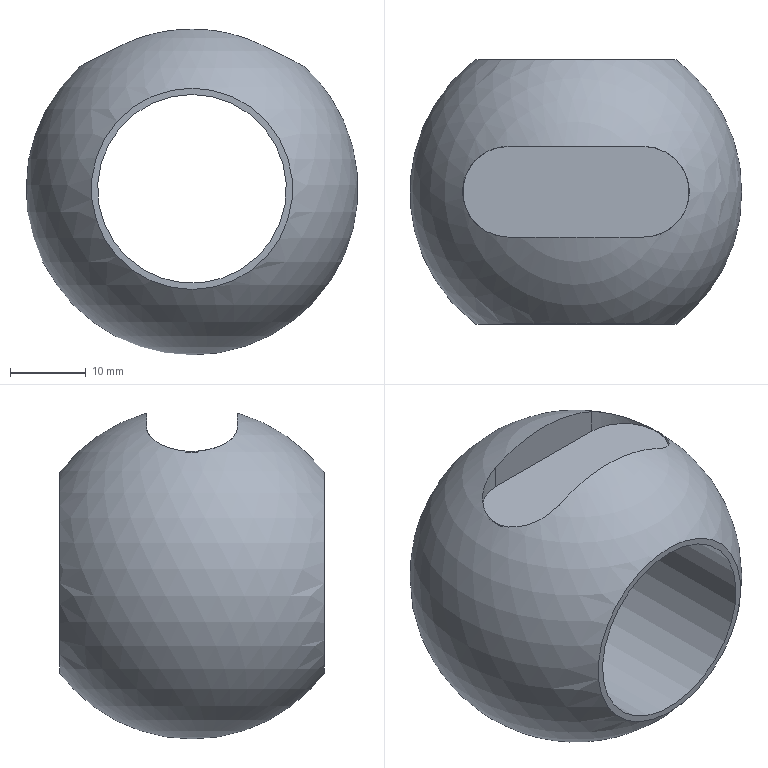Component | NX | VALVECORE | 1 solid | 9 faces | box 44 x 35 x 43.17 mm | volume 23444 mm3 | plane 5 | cylinder 3 | sphere 1 | commonest cylinder face diameters 12 x2 25 x1
STEP:
#1=CARTESIAN_POINT('',(0.,0.,0.));
#2=DIRECTION('',(0.,0.,1.));
#3=DIRECTION('',(1.,0.,0.));
#4=AXIS2_PLACEMENT_3D('',#1,#2,#3);
#5=CARTESIAN_POINT('',(186.165,20.5,51.157));
#6=VERTEX_POINT('',#5);
#7=CARTESIAN_POINT('',(168.165,20.5,51.157));
#8=VERTEX_POINT('',#7);
#9=CARTESIAN_POINT('',(177.165,20.5,32.));
#10=DIRECTION('',(0.,-1.,0.));
#11=DIRECTION('',(0.,0.,1.));
#12=AXIS2_PLACEMENT_3D('',#9,#10,#11);
#13=CIRCLE('',#12,21.166);
#14=CARTESIAN_POINT('',(177.165,26.5,32.));
#15=DIRECTION('',(0.,0.,1.));
#16=DIRECTION('',(1.,0.,0.));
#17=AXIS2_PLACEMENT_3D('',#14,#15,#16);
#18=SPHERICAL_SURFACE('',#17,22.);
#19=CARTESIAN_POINT('',(5.695,1.057));
#20=CARTESIAN_POINT('',(5.682,1.068));
#21=CARTESIAN_POINT('',(5.654,1.09));
#22=CARTESIAN_POINT('',(5.606,1.121));
#23=CARTESIAN_POINT('',(5.55,1.152));
#24=CARTESIAN_POINT('',(5.486,1.181));
#25=CARTESIAN_POINT('',(5.411,1.208));
#26=CARTESIAN_POINT('',(5.325,1.232));
#27=CARTESIAN_POINT('',(5.226,1.253));
#28=CARTESIAN_POINT('',(5.113,1.271));
#29=CARTESIAN_POINT('',(4.988,1.284));
#30=CARTESIAN_POINT('',(4.853,1.293));
#31=CARTESIAN_POINT('',(4.712,1.296));
#32=CARTESIAN_POINT('',(4.572,1.293));
#33=CARTESIAN_POINT('',(4.436,1.284));
#34=CARTESIAN_POINT('',(4.311,1.271));
#35=CARTESIAN_POINT('',(4.199,1.253));
#36=CARTESIAN_POINT('',(4.1,1.232));
#37=CARTESIAN_POINT('',(4.014,1.208));
#38=CARTESIAN_POINT('',(3.939,1.181));
#39=CARTESIAN_POINT('',(3.874,1.152));
#40=CARTESIAN_POINT('',(3.819,1.121));
#41=CARTESIAN_POINT('',(3.771,1.09));
#42=CARTESIAN_POINT('',(3.743,1.068));
#43=CARTESIAN_POINT('',(3.73,1.057));
#44=B_SPLINE_CURVE_WITH_KNOTS('',3,(#19,#20,#21,#22,#23,#24,#25,#26,#27,#28,#29,#30,#31,#32,#33,#34,#35,#36,#37,#38,#39,#40,#41,#42,#43),.UNSPECIFIED.,.F.,.F.,(4,1,1,1,1,1,1,1,1,1,1,1,1,1,1,1,1,1,1,1,1,1,4),(5.844,5.884,5.924,5.964,6.004,6.044,6.084,6.123,6.163,6.203,6.243,6.283,6.323,6.363,6.403,6.443,6.483,6.523,6.563,6.603,6.643,6.682,6.722),.QUASI_UNIFORM_KNOTS.);
#45=(GEOMETRIC_REPRESENTATION_CONTEXT(2)PARAMETRIC_REPRESENTATION_CONTEXT()REPRESENTATION_CONTEXT('',''));
#46=DEFINITIONAL_REPRESENTATION('',(#44),#45);
#47=PCURVE('',#18,#46);
#48=CARTESIAN_POINT('',(168.165,20.5,82.));
#49=DIRECTION('',(0.,1.,0.));
#50=DIRECTION('',(0.,0.,1.));
#51=AXIS2_PLACEMENT_3D('',#48,#49,#50);
#52=PLANE('',#51);
#53=CARTESIAN_POINT('',(-28.834,9.));
#54=CARTESIAN_POINT('',(-28.834,-27.661));
#55=CARTESIAN_POINT('',(-60.583,-9.33));
#56=CARTESIAN_POINT('',(-92.332,9.));
#57=CARTESIAN_POINT('',(-60.583,27.33));
#58=CARTESIAN_POINT('',(-28.834,45.661));
#59=CARTESIAN_POINT('',(-28.834,9.));
#60=(BOUNDED_CURVE()B_SPLINE_CURVE(2,(#53,#54,#55,#56,#57,#58,#59),.UNSPECIFIED.,.T.,.F.)B_SPLINE_CURVE_WITH_KNOTS((1,2,2,2,2,1),(-2.094,0.,2.094,4.189,6.283,8.378),.UNSPECIFIED.)CURVE()GEOMETRIC_REPRESENTATION_ITEM()RATIONAL_B_SPLINE_CURVE((1.,0.5,1.,0.5,1.,0.5,1.))REPRESENTATION_ITEM(''));
#61=(GEOMETRIC_REPRESENTATION_CONTEXT(2)PARAMETRIC_REPRESENTATION_CONTEXT()REPRESENTATION_CONTEXT('',''));
#62=DEFINITIONAL_REPRESENTATION('',(#60),#61);
#63=PCURVE('',#52,#62);
#64=SURFACE_CURVE('',#13,(#47,#63),.PCURVE_S1.);
#65=EDGE_CURVE('',#6,#8,#64,.T.);
#66=ORIENTED_EDGE('',*,*,#65,.T.);
#67=CARTESIAN_POINT('',(168.165,32.5,51.157));
#68=VERTEX_POINT('',#67);
#69=CARTESIAN_POINT('',(168.165,20.5,51.157));
#70=CARTESIAN_POINT('',(166.646,20.5,50.443));
#71=CARTESIAN_POINT('',(165.179,21.065,49.709));
#72=CARTESIAN_POINT('',(162.902,23.221,48.511));
#73=CARTESIAN_POINT('',(162.171,24.818,48.096));
#74=CARTESIAN_POINT('',(162.16,28.145,48.091));
#75=CARTESIAN_POINT('',(162.891,29.763,48.505));
#76=CARTESIAN_POINT('',(165.163,31.927,49.701));
#77=CARTESIAN_POINT('',(166.644,32.5,50.442));
#78=CARTESIAN_POINT('',(168.165,32.5,51.157));
#79=B_SPLINE_CURVE_WITH_KNOTS('',3,(#69,#70,#71,#72,#73,#74,#75,#76,#77,#78),.UNSPECIFIED.,.F.,.F.,(4,2,2,2,4),(0.,0.25,0.5,0.75,1.),.UNSPECIFIED.);
#80=CARTESIAN_POINT('',(3.73,1.057));
#81=CARTESIAN_POINT('',(3.715,1.045));
#82=CARTESIAN_POINT('',(3.686,1.021));
#83=CARTESIAN_POINT('',(3.64,0.9884));
#84=CARTESIAN_POINT('',(3.592,0.9575));
#85=CARTESIAN_POINT('',(3.542,0.9289));
#86=CARTESIAN_POINT('',(3.489,0.9028));
#87=CARTESIAN_POINT('',(3.435,0.8791));
#88=CARTESIAN_POINT('',(3.379,0.859));
#89=CARTESIAN_POINT('',(3.321,0.8426));
#90=CARTESIAN_POINT('',(3.262,0.8303));
#91=CARTESIAN_POINT('',(3.203,0.8225));
#92=CARTESIAN_POINT('',(3.143,0.8196));
#93=CARTESIAN_POINT('',(3.083,0.8223));
#94=CARTESIAN_POINT('',(3.023,0.83));
#95=CARTESIAN_POINT('',(2.964,0.8422));
#96=CARTESIAN_POINT('',(2.906,0.8585));
#97=CARTESIAN_POINT('',(2.849,0.8786));
#98=CARTESIAN_POINT('',(2.795,0.9022));
#99=CARTESIAN_POINT('',(2.742,0.9285));
#100=CARTESIAN_POINT('',(2.692,0.9572));
#101=CARTESIAN_POINT('',(2.643,0.9882));
#102=CARTESIAN_POINT('',(2.597,1.021));
#103=CARTESIAN_POINT('',(2.568,1.045));
#104=CARTESIAN_POINT('',(2.554,1.057));
#105=B_SPLINE_CURVE_WITH_KNOTS('',3,(#80,#81,#82,#83,#84,#85,#86,#87,#88,#89,#90,#91,#92,#93,#94,#95,#96,#97,#98,#99,#100,#101,#102,#103,#104),.UNSPECIFIED.,.F.,.F.,(4,1,1,1,1,1,1,1,1,1,1,1,1,1,1,1,1,1,1,1,1,1,4),(0.,0.04545,0.09091,0.1364,0.1818,0.2273,0.2727,0.3182,0.3636,0.4091,0.4545,0.5,0.5455,0.5909,0.6364,0.6818,0.7273,0.7727,0.8182,0.8636,0.9091,0.9545,1.),.QUASI_UNIFORM_KNOTS.);
#106=(GEOMETRIC_REPRESENTATION_CONTEXT(2)PARAMETRIC_REPRESENTATION_CONTEXT()REPRESENTATION_CONTEXT('',''));
#107=DEFINITIONAL_REPRESENTATION('',(#105),#106);
#108=PCURVE('',#18,#107);
#109=CARTESIAN_POINT('',(168.165,26.5,82.));
#110=DIRECTION('',(0.,0.,-1.));
#111=DIRECTION('',(-1.,0.,0.));
#112=AXIS2_PLACEMENT_3D('',#109,#110,#111);
#113=CYLINDRICAL_SURFACE('',#112,6.);
#114=CARTESIAN_POINT('',(4.712,30.843));
#115=CARTESIAN_POINT('',(4.758,30.973));
#116=CARTESIAN_POINT('',(4.85,31.234));
#117=CARTESIAN_POINT('',(4.986,31.624));
#118=CARTESIAN_POINT('',(5.123,32.006));
#119=CARTESIAN_POINT('',(5.26,32.376));
#120=CARTESIAN_POINT('',(5.399,32.727));
#121=CARTESIAN_POINT('',(5.542,33.056));
#122=CARTESIAN_POINT('',(5.686,33.342));
#123=CARTESIAN_POINT('',(5.833,33.581));
#124=CARTESIAN_POINT('',(5.981,33.762));
#125=CARTESIAN_POINT('',(6.13,33.878));
#126=CARTESIAN_POINT('',(6.28,33.92));
#127=CARTESIAN_POINT('',(6.431,33.88));
#128=CARTESIAN_POINT('',(6.58,33.766));
#129=CARTESIAN_POINT('',(6.729,33.586));
#130=CARTESIAN_POINT('',(6.877,33.349));
#131=CARTESIAN_POINT('',(7.022,33.062));
#132=CARTESIAN_POINT('',(7.164,32.735));
#133=CARTESIAN_POINT('',(7.304,32.383));
#134=CARTESIAN_POINT('',(7.442,32.011));
#135=CARTESIAN_POINT('',(7.579,31.626));
#136=CARTESIAN_POINT('',(7.716,31.234));
#137=CARTESIAN_POINT('',(7.808,30.973));
#138=CARTESIAN_POINT('',(7.854,30.843));
#139=B_SPLINE_CURVE_WITH_KNOTS('',3,(#114,#115,#116,#117,#118,#119,#120,#121,#122,#123,#124,#125,#126,#127,#128,#129,#130,#131,#132,#133,#134,#135,#136,#137,#138),.UNSPECIFIED.,.F.,.F.,(4,1,1,1,1,1,1,1,1,1,1,1,1,1,1,1,1,1,1,1,1,1,4),(0.,0.04545,0.09091,0.1364,0.1818,0.2273,0.2727,0.3182,0.3636,0.4091,0.4545,0.5,0.5455,0.5909,0.6364,0.6818,0.7273,0.7727,0.8182,0.8636,0.9091,0.9545,1.),.QUASI_UNIFORM_KNOTS.);
#140=(GEOMETRIC_REPRESENTATION_CONTEXT(2)PARAMETRIC_REPRESENTATION_CONTEXT()REPRESENTATION_CONTEXT('',''));
#141=DEFINITIONAL_REPRESENTATION('',(#139),#140);
#142=PCURVE('',#113,#141);
#143=SURFACE_CURVE('',#79,(#108,#142),.PCURVE_S1.);
#144=EDGE_CURVE('',#8,#68,#143,.T.);
#145=ORIENTED_EDGE('',*,*,#144,.T.);
#146=CARTESIAN_POINT('',(186.165,32.5,51.157));
#147=VERTEX_POINT('',#146);
#148=CARTESIAN_POINT('',(177.165,32.5,32.));
#149=DIRECTION('',(0.,1.,0.));
#150=DIRECTION('',(0.,0.,-1.));
#151=AXIS2_PLACEMENT_3D('',#148,#149,#150);
#152=CIRCLE('',#151,21.166);
#153=CARTESIAN_POINT('',(2.554,1.057));
#154=CARTESIAN_POINT('',(2.541,1.068));
#155=CARTESIAN_POINT('',(2.513,1.09));
#156=CARTESIAN_POINT('',(2.464,1.121));
#157=CARTESIAN_POINT('',(2.409,1.152));
#158=CARTESIAN_POINT('',(2.344,1.181));
#159=CARTESIAN_POINT('',(2.27,1.208));
#160=CARTESIAN_POINT('',(2.183,1.232));
#161=CARTESIAN_POINT('',(2.084,1.253));
#162=CARTESIAN_POINT('',(1.972,1.271));
#163=CARTESIAN_POINT('',(1.847,1.284));
#164=CARTESIAN_POINT('',(1.712,1.293));
#165=CARTESIAN_POINT('',(1.571,1.296));
#166=CARTESIAN_POINT('',(1.43,1.293));
#167=CARTESIAN_POINT('',(1.295,1.284));
#168=CARTESIAN_POINT('',(1.17,1.271));
#169=CARTESIAN_POINT('',(1.057,1.253));
#170=CARTESIAN_POINT('',(0.9582,1.232));
#171=CARTESIAN_POINT('',(0.8719,1.208));
#172=CARTESIAN_POINT('',(0.7973,1.181));
#173=CARTESIAN_POINT('',(0.7329,1.152));
#174=CARTESIAN_POINT('',(0.6772,1.121));
#175=CARTESIAN_POINT('',(0.629,1.09));
#176=CARTESIAN_POINT('',(0.6011,1.068));
#177=CARTESIAN_POINT('',(0.588,1.057));
#178=B_SPLINE_CURVE_WITH_KNOTS('',3,(#153,#154,#155,#156,#157,#158,#159,#160,#161,#162,#163,#164,#165,#166,#167,#168,#169,#170,#171,#172,#173,#174,#175,#176,#177),.UNSPECIFIED.,.F.,.F.,(4,1,1,1,1,1,1,1,1,1,1,1,1,1,1,1,1,1,1,1,1,1,4),(2.702,2.742,2.782,2.822,2.862,2.902,2.942,2.982,3.022,3.062,3.102,3.142,3.182,3.221,3.261,3.301,3.341,3.381,3.421,3.461,3.501,3.541,3.581),.QUASI_UNIFORM_KNOTS.);
#179=(GEOMETRIC_REPRESENTATION_CONTEXT(2)PARAMETRIC_REPRESENTATION_CONTEXT()REPRESENTATION_CONTEXT('',''));
#180=DEFINITIONAL_REPRESENTATION('',(#178),#179);
#181=PCURVE('',#18,#180);
#182=CARTESIAN_POINT('',(186.165,32.5,82.));
#183=DIRECTION('',(0.,-1.,0.));
#184=DIRECTION('',(0.,0.,-1.));
#185=AXIS2_PLACEMENT_3D('',#182,#183,#184);
#186=PLANE('',#185);
#187=CARTESIAN_POINT('',(71.166,-9.));
#188=CARTESIAN_POINT('',(71.166,-45.661));
#189=CARTESIAN_POINT('',(39.417,-27.33));
#190=CARTESIAN_POINT('',(7.668,-9.));
#191=CARTESIAN_POINT('',(39.417,9.33));
#192=CARTESIAN_POINT('',(71.166,27.661));
#193=CARTESIAN_POINT('',(71.166,-9.));
#194=(BOUNDED_CURVE()B_SPLINE_CURVE(2,(#187,#188,#189,#190,#191,#192,#193),.UNSPECIFIED.,.T.,.F.)B_SPLINE_CURVE_WITH_KNOTS((1,2,2,2,2,1),(-2.094,0.,2.094,4.189,6.283,8.378),.UNSPECIFIED.)CURVE()GEOMETRIC_REPRESENTATION_ITEM()RATIONAL_B_SPLINE_CURVE((1.,0.5,1.,0.5,1.,0.5,1.))REPRESENTATION_ITEM(''));
#195=(GEOMETRIC_REPRESENTATION_CONTEXT(2)PARAMETRIC_REPRESENTATION_CONTEXT()REPRESENTATION_CONTEXT('',''));
#196=DEFINITIONAL_REPRESENTATION('',(#194),#195);
#197=PCURVE('',#186,#196);
#198=SURFACE_CURVE('',#152,(#181,#197),.PCURVE_S1.);
#199=EDGE_CURVE('',#68,#147,#198,.T.);
#200=ORIENTED_EDGE('',*,*,#199,.T.);
#201=CARTESIAN_POINT('',(192.165,26.5,48.093));
#202=VERTEX_POINT('',#201);
#203=CARTESIAN_POINT('',(186.165,32.5,51.157));
#204=CARTESIAN_POINT('',(187.685,32.5,50.443));
#205=CARTESIAN_POINT('',(189.152,31.935,49.709));
#206=CARTESIAN_POINT('',(191.429,29.779,48.511));
#207=CARTESIAN_POINT('',(192.16,28.182,48.096));
#208=CARTESIAN_POINT('',(192.17,24.855,48.091));
#209=CARTESIAN_POINT('',(191.44,23.237,48.505));
#210=CARTESIAN_POINT('',(189.168,21.073,49.701));
#211=CARTESIAN_POINT('',(187.687,20.5,50.442));
#212=CARTESIAN_POINT('',(186.165,20.5,51.157));
#213=B_SPLINE_CURVE_WITH_KNOTS('',3,(#203,#204,#205,#206,#207,#208,#209,#210,#211,#212),.UNSPECIFIED.,.F.,.F.,(4,2,2,2,4),(0.,0.25,0.5,0.75,1.),.UNSPECIFIED.);
#214=CARTESIAN_POINT('',(0.588,1.057));
#215=CARTESIAN_POINT('',(0.5738,1.045));
#216=CARTESIAN_POINT('',(0.5446,1.021));
#217=CARTESIAN_POINT('',(0.4985,0.9884));
#218=CARTESIAN_POINT('',(0.4503,0.9575));
#219=CARTESIAN_POINT('',(0.4001,0.9289));
#220=CARTESIAN_POINT('',(0.3479,0.9028));
#221=CARTESIAN_POINT('',(0.2933,0.8791));
#222=CARTESIAN_POINT('',(0.237,0.859));
#223=CARTESIAN_POINT('',(0.1794,0.8426));
#224=CARTESIAN_POINT('',(0.1208,0.8303));
#225=CARTESIAN_POINT('',(0.06147,0.8225));
#226=CARTESIAN_POINT('',(0.001252,0.8196));
#227=CARTESIAN_POINT('',(-0.05907,0.8223));
#228=CARTESIAN_POINT('',(-0.1186,0.83));
#229=CARTESIAN_POINT('',(-0.1776,0.8422));
#230=CARTESIAN_POINT('',(-0.2355,0.8585));
#231=CARTESIAN_POINT('',(-0.2922,0.8786));
#232=CARTESIAN_POINT('',(-0.3467,0.9022));
#233=CARTESIAN_POINT('',(-0.3991,0.9285));
#234=CARTESIAN_POINT('',(-0.4496,0.9572));
#235=CARTESIAN_POINT('',(-0.4981,0.9882));
#236=CARTESIAN_POINT('',(-0.5445,1.021));
#237=CARTESIAN_POINT('',(-0.5738,1.045));
#238=CARTESIAN_POINT('',(-0.588,1.057));
#239=B_SPLINE_CURVE_WITH_KNOTS('',3,(#214,#215,#216,#217,#218,#219,#220,#221,#222,#223,#224,#225,#226,#227,#228,#229,#230,#231,#232,#233,#234,#235,#236,#237,#238),.UNSPECIFIED.,.F.,.F.,(4,1,1,1,1,1,1,1,1,1,1,1,1,1,1,1,1,1,1,1,1,1,4),(0.,0.04545,0.09091,0.1364,0.1818,0.2273,0.2727,0.3182,0.3636,0.4091,0.4545,0.5,0.5455,0.5909,0.6364,0.6818,0.7273,0.7727,0.8182,0.8636,0.9091,0.9545,1.),.QUASI_UNIFORM_KNOTS.);
#240=(GEOMETRIC_REPRESENTATION_CONTEXT(2)PARAMETRIC_REPRESENTATION_CONTEXT()REPRESENTATION_CONTEXT('',''));
#241=DEFINITIONAL_REPRESENTATION('',(#239),#240);
#242=PCURVE('',#18,#241);
#243=CARTESIAN_POINT('',(186.165,26.5,82.));
#244=DIRECTION('',(0.,0.,-1.));
#245=DIRECTION('',(-1.,0.,0.));
#246=AXIS2_PLACEMENT_3D('',#243,#244,#245);
#247=CYLINDRICAL_SURFACE('',#246,6.);
#248=CARTESIAN_POINT('',(1.571,30.843));
#249=CARTESIAN_POINT('',(1.594,30.908));
#250=CARTESIAN_POINT('',(1.64,31.038));
#251=CARTESIAN_POINT('',(1.709,31.234));
#252=CARTESIAN_POINT('',(1.777,31.43));
#253=CARTESIAN_POINT('',(1.845,31.624));
#254=CARTESIAN_POINT('',(1.914,31.817));
#255=CARTESIAN_POINT('',(1.982,32.007));
#256=CARTESIAN_POINT('',(2.051,32.194));
#257=CARTESIAN_POINT('',(2.12,32.377));
#258=CARTESIAN_POINT('',(2.189,32.555));
#259=CARTESIAN_POINT('',(2.259,32.728));
#260=CARTESIAN_POINT('',(2.33,32.895));
#261=CARTESIAN_POINT('',(2.402,33.054));
#262=CARTESIAN_POINT('',(2.474,33.202));
#263=CARTESIAN_POINT('',(2.547,33.34));
#264=CARTESIAN_POINT('',(2.62,33.465));
#265=CARTESIAN_POINT('',(2.693,33.577));
#266=CARTESIAN_POINT('',(2.767,33.674));
#267=CARTESIAN_POINT('',(2.842,33.756));
#268=CARTESIAN_POINT('',(2.916,33.822));
#269=CARTESIAN_POINT('',(2.991,33.87));
#270=CARTESIAN_POINT('',(3.066,33.9));
#271=CARTESIAN_POINT('',(3.116,33.907));
#272=CARTESIAN_POINT('',(3.142,33.907));
#273=B_SPLINE_CURVE_WITH_KNOTS('',3,(#248,#249,#250,#251,#252,#253,#254,#255,#256,#257,#258,#259,#260,#261,#262,#263,#264,#265,#266,#267,#268,#269,#270,#271,#272),.UNSPECIFIED.,.F.,.F.,(4,1,1,1,1,1,1,1,1,1,1,1,1,1,1,1,1,1,1,1,1,1,4),(0.,0.02277,0.04554,0.06831,0.09108,0.1138,0.1366,0.1594,0.1822,0.2049,0.2277,0.2505,0.2732,0.296,0.3188,0.3415,0.3643,0.3871,0.4099,0.4326,0.4554,0.4782,0.5009),.QUASI_UNIFORM_KNOTS.);
#274=(GEOMETRIC_REPRESENTATION_CONTEXT(2)PARAMETRIC_REPRESENTATION_CONTEXT()REPRESENTATION_CONTEXT('',''));
#275=DEFINITIONAL_REPRESENTATION('',(#273),#274);
#276=PCURVE('',#247,#275);
#277=SURFACE_CURVE('',#213,(#242,#276),.PCURVE_S1.);
#278=EDGE_CURVE('',#147,#202,#277,.T.);
#279=ORIENTED_EDGE('',*,*,#278,.T.);
#280=CARTESIAN_POINT('',(177.165,26.5,10.));
#281=VERTEX_POINT('',#280);
#282=CARTESIAN_POINT('',(177.165,26.5,10.));
#283=CARTESIAN_POINT('',(183.742,26.5,10.));
#284=CARTESIAN_POINT('',(190.318,26.5,12.247));
#285=CARTESIAN_POINT('',(195.998,26.5,16.739));
#286=CARTESIAN_POINT('',(199.889,26.5,23.052));
#287=CARTESIAN_POINT('',(201.347,26.5,30.323));
#288=CARTESIAN_POINT('',(200.255,26.5,37.482));
#289=CARTESIAN_POINT('',(196.976,26.5,43.61));
#290=CARTESIAN_POINT('',(192.165,26.5,48.093));
#291=B_SPLINE_CURVE_WITH_KNOTS('',8,(#282,#283,#284,#285,#286,#287,#288,#289,#290),.UNSPECIFIED.,.F.,.F.,(9,9),(-1.571,0.8206),.PIECEWISE_BEZIER_KNOTS.);
#292=CARTESIAN_POINT('',(0.,0.));
#293=DIRECTION('',(0.,1.));
#294=VECTOR('',#293,1.);
#295=LINE('',#292,#294);
#296=(GEOMETRIC_REPRESENTATION_CONTEXT(2)PARAMETRIC_REPRESENTATION_CONTEXT()REPRESENTATION_CONTEXT('',''));
#297=DEFINITIONAL_REPRESENTATION('',(#295),#296);
#298=PCURVE('',#18,#297);
#299=CARTESIAN_POINT('',(6.283,0.));
#300=DIRECTION('',(0.,1.));
#301=VECTOR('',#300,1.);
#302=LINE('',#299,#301);
#303=(GEOMETRIC_REPRESENTATION_CONTEXT(2)PARAMETRIC_REPRESENTATION_CONTEXT()REPRESENTATION_CONTEXT('',''));
#304=DEFINITIONAL_REPRESENTATION('',(#302),#303);
#305=PCURVE('',#18,#304);
#306=SEAM_CURVE('',#291,(#298,#305),.PCURVE_S1.);
#307=EDGE_CURVE('',#281,#202,#306,.T.);
#308=ORIENTED_EDGE('',*,*,#307,.F.);
#309=ORIENTED_EDGE('',*,*,#307,.T.);
#310=CARTESIAN_POINT('',(186.165,32.5,51.157));
#311=CARTESIAN_POINT('',(187.685,32.5,50.443));
#312=CARTESIAN_POINT('',(189.152,31.935,49.709));
#313=CARTESIAN_POINT('',(191.429,29.779,48.511));
#314=CARTESIAN_POINT('',(192.16,28.182,48.096));
#315=CARTESIAN_POINT('',(192.17,24.855,48.091));
#316=CARTESIAN_POINT('',(191.44,23.237,48.505));
#317=CARTESIAN_POINT('',(189.168,21.073,49.701));
#318=CARTESIAN_POINT('',(187.687,20.5,50.442));
#319=CARTESIAN_POINT('',(186.165,20.5,51.157));
#320=B_SPLINE_CURVE_WITH_KNOTS('',3,(#310,#311,#312,#313,#314,#315,#316,#317,#318,#319),.UNSPECIFIED.,.F.,.F.,(4,2,2,2,4),(0.,0.25,0.5,0.75,1.),.UNSPECIFIED.);
#321=CARTESIAN_POINT('',(6.871,1.057));
#322=CARTESIAN_POINT('',(6.857,1.045));
#323=CARTESIAN_POINT('',(6.828,1.021));
#324=CARTESIAN_POINT('',(6.782,0.9884));
#325=CARTESIAN_POINT('',(6.733,0.9575));
#326=CARTESIAN_POINT('',(6.683,0.9289));
#327=CARTESIAN_POINT('',(6.631,0.9028));
#328=CARTESIAN_POINT('',(6.577,0.8791));
#329=CARTESIAN_POINT('',(6.52,0.859));
#330=CARTESIAN_POINT('',(6.463,0.8426));
#331=CARTESIAN_POINT('',(6.404,0.8303));
#332=CARTESIAN_POINT('',(6.345,0.8225));
#333=CARTESIAN_POINT('',(6.284,0.8196));
#334=CARTESIAN_POINT('',(6.224,0.8223));
#335=CARTESIAN_POINT('',(6.165,0.83));
#336=CARTESIAN_POINT('',(6.106,0.8422));
#337=CARTESIAN_POINT('',(6.048,0.8585));
#338=CARTESIAN_POINT('',(5.991,0.8786));
#339=CARTESIAN_POINT('',(5.936,0.9022));
#340=CARTESIAN_POINT('',(5.884,0.9285));
#341=CARTESIAN_POINT('',(5.834,0.9572));
#342=CARTESIAN_POINT('',(5.785,0.9882));
#343=CARTESIAN_POINT('',(5.739,1.021));
#344=CARTESIAN_POINT('',(5.709,1.045));
#345=CARTESIAN_POINT('',(5.695,1.057));
#346=B_SPLINE_CURVE_WITH_KNOTS('',3,(#321,#322,#323,#324,#325,#326,#327,#328,#329,#330,#331,#332,#333,#334,#335,#336,#337,#338,#339,#340,#341,#342,#343,#344,#345),.UNSPECIFIED.,.F.,.F.,(4,1,1,1,1,1,1,1,1,1,1,1,1,1,1,1,1,1,1,1,1,1,4),(0.,0.04545,0.09091,0.1364,0.1818,0.2273,0.2727,0.3182,0.3636,0.4091,0.4545,0.5,0.5455,0.5909,0.6364,0.6818,0.7273,0.7727,0.8182,0.8636,0.9091,0.9545,1.),.QUASI_UNIFORM_KNOTS.);
#347=(GEOMETRIC_REPRESENTATION_CONTEXT(2)PARAMETRIC_REPRESENTATION_CONTEXT()REPRESENTATION_CONTEXT('',''));
#348=DEFINITIONAL_REPRESENTATION('',(#346),#347);
#349=PCURVE('',#18,#348);
#350=CARTESIAN_POINT('',(3.142,33.907));
#351=CARTESIAN_POINT('',(3.167,33.907));
#352=CARTESIAN_POINT('',(3.217,33.9));
#353=CARTESIAN_POINT('',(3.292,33.87));
#354=CARTESIAN_POINT('',(3.367,33.821));
#355=CARTESIAN_POINT('',(3.441,33.756));
#356=CARTESIAN_POINT('',(3.516,33.673));
#357=CARTESIAN_POINT('',(3.59,33.576));
#358=CARTESIAN_POINT('',(3.663,33.464));
#359=CARTESIAN_POINT('',(3.737,33.339));
#360=CARTESIAN_POINT('',(3.809,33.202));
#361=CARTESIAN_POINT('',(3.881,33.054));
#362=CARTESIAN_POINT('',(3.953,32.895));
#363=CARTESIAN_POINT('',(4.024,32.728));
#364=CARTESIAN_POINT('',(4.094,32.556));
#365=CARTESIAN_POINT('',(4.163,32.377));
#366=CARTESIAN_POINT('',(4.232,32.194));
#367=CARTESIAN_POINT('',(4.301,32.007));
#368=CARTESIAN_POINT('',(4.37,31.817));
#369=CARTESIAN_POINT('',(4.438,31.624));
#370=CARTESIAN_POINT('',(4.506,31.429));
#371=CARTESIAN_POINT('',(4.575,31.234));
#372=CARTESIAN_POINT('',(4.643,31.038));
#373=CARTESIAN_POINT('',(4.689,30.908));
#374=CARTESIAN_POINT('',(4.712,30.843));
#375=B_SPLINE_CURVE_WITH_KNOTS('',3,(#350,#351,#352,#353,#354,#355,#356,#357,#358,#359,#360,#361,#362,#363,#364,#365,#366,#367,#368,#369,#370,#371,#372,#373,#374),.UNSPECIFIED.,.F.,.F.,(4,1,1,1,1,1,1,1,1,1,1,1,1,1,1,1,1,1,1,1,1,1,4),(0.5009,0.5236,0.5463,0.569,0.5917,0.6144,0.637,0.6597,0.6824,0.7051,0.7278,0.7505,0.7732,0.7958,0.8185,0.8412,0.8639,0.8866,0.9093,0.9319,0.9546,0.9773,1.),.QUASI_UNIFORM_KNOTS.);
#376=(GEOMETRIC_REPRESENTATION_CONTEXT(2)PARAMETRIC_REPRESENTATION_CONTEXT()REPRESENTATION_CONTEXT('',''));
#377=DEFINITIONAL_REPRESENTATION('',(#375),#376);
#378=PCURVE('',#247,#377);
#379=SURFACE_CURVE('',#320,(#349,#378),.PCURVE_S1.);
#380=EDGE_CURVE('',#202,#6,#379,.T.);
#381=ORIENTED_EDGE('',*,*,#380,.T.);
#382=EDGE_LOOP('',(#66,#145,#200,#279,#308,#309,#381));
#383=FACE_BOUND('',#382,.T.);
#384=CARTESIAN_POINT('',(177.165,44.,45.332));
#385=VERTEX_POINT('',#384);
#386=CARTESIAN_POINT('',(177.165,44.,32.));
#387=DIRECTION('',(0.,-1.,0.));
#388=DIRECTION('',(0.,0.,1.));
#389=AXIS2_PLACEMENT_3D('',#386,#387,#388);
#390=CIRCLE('',#389,13.332);
#391=CARTESIAN_POINT('',(1.571,0.651));
#392=CARTESIAN_POINT('',(1.645,0.6516));
#393=CARTESIAN_POINT('',(1.787,0.6297));
#394=CARTESIAN_POINT('',(1.97,0.5419));
#395=CARTESIAN_POINT('',(2.101,0.4124));
#396=CARTESIAN_POINT('',(2.184,0.2568));
#397=CARTESIAN_POINT('',(2.223,0.08709));
#398=CARTESIAN_POINT('',(2.223,-0.08709));
#399=CARTESIAN_POINT('',(2.184,-0.2568));
#400=CARTESIAN_POINT('',(2.101,-0.4125));
#401=CARTESIAN_POINT('',(1.97,-0.5418));
#402=CARTESIAN_POINT('',(1.788,-0.6299));
#403=CARTESIAN_POINT('',(1.571,-0.6616));
#404=CARTESIAN_POINT('',(1.353,-0.6299));
#405=CARTESIAN_POINT('',(1.172,-0.5418));
#406=CARTESIAN_POINT('',(1.04,-0.4125));
#407=CARTESIAN_POINT('',(0.9576,-0.2568));
#408=CARTESIAN_POINT('',(0.9181,-0.08709));
#409=CARTESIAN_POINT('',(0.9181,0.08709));
#410=CARTESIAN_POINT('',(0.9576,0.2568));
#411=CARTESIAN_POINT('',(1.04,0.4124));
#412=CARTESIAN_POINT('',(1.172,0.5419));
#413=CARTESIAN_POINT('',(1.354,0.6297));
#414=CARTESIAN_POINT('',(1.497,0.6516));
#415=CARTESIAN_POINT('',(1.571,0.651));
#416=B_SPLINE_CURVE_WITH_KNOTS('',3,(#391,#392,#393,#394,#395,#396,#397,#398,#399,#400,#401,#402,#403,#404,#405,#406,#407,#408,#409,#410,#411,#412,#413,#414,#415),.UNSPECIFIED.,.T.,.F.,(4,1,1,1,1,1,1,1,1,1,1,1,1,1,1,1,1,1,1,1,1,1,4),(0.,0.2856,0.5712,0.8568,1.142,1.428,1.714,1.999,2.285,2.57,2.856,3.142,3.427,3.713,3.998,4.284,4.57,4.855,5.141,5.426,5.712,5.998,6.283),.QUASI_UNIFORM_KNOTS.);
#417=(GEOMETRIC_REPRESENTATION_CONTEXT(2)PARAMETRIC_REPRESENTATION_CONTEXT()REPRESENTATION_CONTEXT('',''));
#418=DEFINITIONAL_REPRESENTATION('',(#416),#417);
#419=PCURVE('',#18,#418);
#420=CARTESIAN_POINT('',(177.165,44.,32.));
#421=DIRECTION('',(0.,1.,0.));
#422=DIRECTION('',(0.,0.,1.));
#423=AXIS2_PLACEMENT_3D('',#420,#421,#422);
#424=PLANE('',#423);
#425=CARTESIAN_POINT('',(13.332,0.));
#426=CARTESIAN_POINT('',(13.332,-23.092));
#427=CARTESIAN_POINT('',(-6.666,-11.546));
#428=CARTESIAN_POINT('',(-26.665,-0.));
#429=CARTESIAN_POINT('',(-6.666,11.546));
#430=CARTESIAN_POINT('',(13.332,23.092));
#431=CARTESIAN_POINT('',(13.332,0.));
#432=(BOUNDED_CURVE()B_SPLINE_CURVE(2,(#425,#426,#427,#428,#429,#430,#431),.UNSPECIFIED.,.T.,.F.)B_SPLINE_CURVE_WITH_KNOTS((1,2,2,2,2,1),(-2.094,0.,2.094,4.189,6.283,8.378),.UNSPECIFIED.)CURVE()GEOMETRIC_REPRESENTATION_ITEM()RATIONAL_B_SPLINE_CURVE((1.,0.5,1.,0.5,1.,0.5,1.))REPRESENTATION_ITEM(''));
#433=(GEOMETRIC_REPRESENTATION_CONTEXT(2)PARAMETRIC_REPRESENTATION_CONTEXT()REPRESENTATION_CONTEXT('',''));
#434=DEFINITIONAL_REPRESENTATION('',(#432),#433);
#435=PCURVE('',#424,#434);
#436=SURFACE_CURVE('',#390,(#419,#435),.PCURVE_S1.);
#437=EDGE_CURVE('',#385,#385,#436,.T.);
#438=ORIENTED_EDGE('',*,*,#437,.T.);
#439=EDGE_LOOP('',(#438));
#440=FACE_BOUND('',#439,.T.);
#441=CARTESIAN_POINT('',(177.165,9.,18.668));
#442=VERTEX_POINT('',#441);
#443=CARTESIAN_POINT('',(177.165,9.,32.));
#444=DIRECTION('',(0.,1.,0.));
#445=DIRECTION('',(0.,0.,-1.));
#446=AXIS2_PLACEMENT_3D('',#443,#444,#445);
#447=CIRCLE('',#446,13.332);
#448=CARTESIAN_POINT('',(4.712,-0.651));
#449=CARTESIAN_POINT('',(4.638,-0.6516));
#450=CARTESIAN_POINT('',(4.496,-0.6297));
#451=CARTESIAN_POINT('',(4.313,-0.5419));
#452=CARTESIAN_POINT('',(4.182,-0.4124));
#453=CARTESIAN_POINT('',(4.099,-0.2568));
#454=CARTESIAN_POINT('',(4.06,-0.08709));
#455=CARTESIAN_POINT('',(4.06,0.08709));
#456=CARTESIAN_POINT('',(4.099,0.2568));
#457=CARTESIAN_POINT('',(4.182,0.4125));
#458=CARTESIAN_POINT('',(4.313,0.5418));
#459=CARTESIAN_POINT('',(4.495,0.6299));
#460=CARTESIAN_POINT('',(4.712,0.6616));
#461=CARTESIAN_POINT('',(4.93,0.6299));
#462=CARTESIAN_POINT('',(5.111,0.5418));
#463=CARTESIAN_POINT('',(5.243,0.4125));
#464=CARTESIAN_POINT('',(5.326,0.2568));
#465=CARTESIAN_POINT('',(5.365,0.08709));
#466=CARTESIAN_POINT('',(5.365,-0.08709));
#467=CARTESIAN_POINT('',(5.326,-0.2568));
#468=CARTESIAN_POINT('',(5.243,-0.4124));
#469=CARTESIAN_POINT('',(5.112,-0.5419));
#470=CARTESIAN_POINT('',(4.929,-0.6297));
#471=CARTESIAN_POINT('',(4.787,-0.6516));
#472=CARTESIAN_POINT('',(4.712,-0.651));
#473=B_SPLINE_CURVE_WITH_KNOTS('',3,(#448,#449,#450,#451,#452,#453,#454,#455,#456,#457,#458,#459,#460,#461,#462,#463,#464,#465,#466,#467,#468,#469,#470,#471,#472),.UNSPECIFIED.,.T.,.F.,(4,1,1,1,1,1,1,1,1,1,1,1,1,1,1,1,1,1,1,1,1,1,4),(0.,0.2856,0.5712,0.8568,1.142,1.428,1.714,1.999,2.285,2.57,2.856,3.142,3.427,3.713,3.998,4.284,4.57,4.855,5.141,5.426,5.712,5.998,6.283),.QUASI_UNIFORM_KNOTS.);
#474=(GEOMETRIC_REPRESENTATION_CONTEXT(2)PARAMETRIC_REPRESENTATION_CONTEXT()REPRESENTATION_CONTEXT('',''));
#475=DEFINITIONAL_REPRESENTATION('',(#473),#474);
#476=PCURVE('',#18,#475);
#477=CARTESIAN_POINT('',(177.165,9.,32.));
#478=DIRECTION('',(0.,-1.,0.));
#479=DIRECTION('',(0.,0.,-1.));
#480=AXIS2_PLACEMENT_3D('',#477,#478,#479);
#481=PLANE('',#480);
#482=CARTESIAN_POINT('',(13.332,0.));
#483=CARTESIAN_POINT('',(13.332,-23.092));
#484=CARTESIAN_POINT('',(-6.666,-11.546));
#485=CARTESIAN_POINT('',(-26.665,-0.));
#486=CARTESIAN_POINT('',(-6.666,11.546));
#487=CARTESIAN_POINT('',(13.332,23.092));
#488=CARTESIAN_POINT('',(13.332,0.));
#489=(BOUNDED_CURVE()B_SPLINE_CURVE(2,(#482,#483,#484,#485,#486,#487,#488),.UNSPECIFIED.,.T.,.F.)B_SPLINE_CURVE_WITH_KNOTS((1,2,2,2,2,1),(-2.094,0.,2.094,4.189,6.283,8.378),.UNSPECIFIED.)CURVE()GEOMETRIC_REPRESENTATION_ITEM()RATIONAL_B_SPLINE_CURVE((1.,0.5,1.,0.5,1.,0.5,1.))REPRESENTATION_ITEM(''));
#490=(GEOMETRIC_REPRESENTATION_CONTEXT(2)PARAMETRIC_REPRESENTATION_CONTEXT()REPRESENTATION_CONTEXT('',''));
#491=DEFINITIONAL_REPRESENTATION('',(#489),#490);
#492=PCURVE('',#481,#491);
#493=SURFACE_CURVE('',#447,(#476,#492),.PCURVE_S1.);
#494=EDGE_CURVE('',#442,#442,#493,.T.);
#495=ORIENTED_EDGE('',*,*,#494,.T.);
#496=EDGE_LOOP('',(#495));
#497=FACE_BOUND('',#496,.T.);
#498=ADVANCED_FACE('',(#383,#440,#497),#18,.T.);
#499=CARTESIAN_POINT('',(177.165,44.,44.5));
#500=VERTEX_POINT('',#499);
#501=CARTESIAN_POINT('',(177.165,44.,32.));
#502=DIRECTION('',(0.,1.,0.));
#503=DIRECTION('',(0.,0.,1.));
#504=AXIS2_PLACEMENT_3D('',#501,#502,#503);
#505=CIRCLE('',#504,12.5);
#506=CARTESIAN_POINT('',(0.,0.));
#507=DIRECTION('',(1.,0.));
#508=AXIS2_PLACEMENT_2D('',#506,#507);
#509=CIRCLE('',#508,12.5);
#510=(GEOMETRIC_REPRESENTATION_CONTEXT(2)PARAMETRIC_REPRESENTATION_CONTEXT()REPRESENTATION_CONTEXT('',''));
#511=DEFINITIONAL_REPRESENTATION('',(#509),#510);
#512=PCURVE('',#424,#511);
#513=CARTESIAN_POINT('',(177.165,9.,32.));
#514=DIRECTION('',(0.,1.,0.));
#515=DIRECTION('',(0.,0.,1.));
#516=AXIS2_PLACEMENT_3D('',#513,#514,#515);
#517=CYLINDRICAL_SURFACE('',#516,12.5);
#518=CARTESIAN_POINT('',(0.,35.));
#519=DIRECTION('',(1.,0.));
#520=VECTOR('',#519,1.);
#521=LINE('',#518,#520);
#522=(GEOMETRIC_REPRESENTATION_CONTEXT(2)PARAMETRIC_REPRESENTATION_CONTEXT()REPRESENTATION_CONTEXT('',''));
#523=DEFINITIONAL_REPRESENTATION('',(#521),#522);
#524=PCURVE('',#517,#523);
#525=SURFACE_CURVE('',#505,(#512,#524),.PCURVE_S1.);
#526=EDGE_CURVE('',#500,#500,#525,.T.);
#527=ORIENTED_EDGE('',*,*,#526,.F.);
#528=EDGE_LOOP('',(#527));
#529=FACE_BOUND('',#528,.T.);
#530=ORIENTED_EDGE('',*,*,#437,.F.);
#531=EDGE_LOOP('',(#530));
#532=FACE_BOUND('',#531,.T.);
#533=ADVANCED_FACE('',(#529,#532),#424,.T.);
#534=CARTESIAN_POINT('',(177.165,9.,44.5));
#535=VERTEX_POINT('',#534);
#536=CARTESIAN_POINT('',(177.165,9.,32.));
#537=DIRECTION('',(0.,1.,0.));
#538=DIRECTION('',(0.,0.,1.));
#539=AXIS2_PLACEMENT_3D('',#536,#537,#538);
#540=CIRCLE('',#539,12.5);
#541=CARTESIAN_POINT('',(-12.5,0.));
#542=CARTESIAN_POINT('',(-12.5,21.651));
#543=CARTESIAN_POINT('',(6.25,10.825));
#544=CARTESIAN_POINT('',(25.,0.));
#545=CARTESIAN_POINT('',(6.25,-10.825));
#546=CARTESIAN_POINT('',(-12.5,-21.651));
#547=CARTESIAN_POINT('',(-12.5,0.));
#548=(BOUNDED_CURVE()B_SPLINE_CURVE(2,(#541,#542,#543,#544,#545,#546,#547),.UNSPECIFIED.,.T.,.F.)B_SPLINE_CURVE_WITH_KNOTS((1,2,2,2,2,1),(-2.094,0.,2.094,4.189,6.283,8.378),.UNSPECIFIED.)CURVE()GEOMETRIC_REPRESENTATION_ITEM()RATIONAL_B_SPLINE_CURVE((1.,0.5,1.,0.5,1.,0.5,1.))REPRESENTATION_ITEM(''));
#549=(GEOMETRIC_REPRESENTATION_CONTEXT(2)PARAMETRIC_REPRESENTATION_CONTEXT()REPRESENTATION_CONTEXT('',''));
#550=DEFINITIONAL_REPRESENTATION('',(#548),#549);
#551=PCURVE('',#481,#550);
#552=CARTESIAN_POINT('',(0.,0.));
#553=DIRECTION('',(1.,0.));
#554=VECTOR('',#553,1.);
#555=LINE('',#552,#554);
#556=(GEOMETRIC_REPRESENTATION_CONTEXT(2)PARAMETRIC_REPRESENTATION_CONTEXT()REPRESENTATION_CONTEXT('',''));
#557=DEFINITIONAL_REPRESENTATION('',(#555),#556);
#558=PCURVE('',#517,#557);
#559=SURFACE_CURVE('',#540,(#551,#558),.PCURVE_S1.);
#560=EDGE_CURVE('',#535,#535,#559,.T.);
#561=ORIENTED_EDGE('',*,*,#560,.T.);
#562=EDGE_LOOP('',(#561));
#563=FACE_BOUND('',#562,.T.);
#564=ORIENTED_EDGE('',*,*,#494,.F.);
#565=EDGE_LOOP('',(#564));
#566=FACE_BOUND('',#565,.T.);
#567=ADVANCED_FACE('',(#563,#566),#481,.T.);
#568=ORIENTED_EDGE('',*,*,#526,.F.);
#569=CARTESIAN_POINT('',(177.165,9.,44.5));
#570=CARTESIAN_POINT('',(177.165,44.,44.5));
#571=B_SPLINE_CURVE_WITH_KNOTS('',1,(#569,#570),.UNSPECIFIED.,.F.,.F.,(2,2),(0.,35.),.PIECEWISE_BEZIER_KNOTS.);
#572=CARTESIAN_POINT('',(0.,0.));
#573=DIRECTION('',(0.,1.));
#574=VECTOR('',#573,1.);
#575=LINE('',#572,#574);
#576=(GEOMETRIC_REPRESENTATION_CONTEXT(2)PARAMETRIC_REPRESENTATION_CONTEXT()REPRESENTATION_CONTEXT('',''));
#577=DEFINITIONAL_REPRESENTATION('',(#575),#576);
#578=PCURVE('',#517,#577);
#579=CARTESIAN_POINT('',(6.283,0.));
#580=DIRECTION('',(0.,1.));
#581=VECTOR('',#580,1.);
#582=LINE('',#579,#581);
#583=(GEOMETRIC_REPRESENTATION_CONTEXT(2)PARAMETRIC_REPRESENTATION_CONTEXT()REPRESENTATION_CONTEXT('',''));
#584=DEFINITIONAL_REPRESENTATION('',(#582),#583);
#585=PCURVE('',#517,#584);
#586=SEAM_CURVE('',#571,(#578,#585),.PCURVE_S1.);
#587=EDGE_CURVE('',#535,#500,#586,.T.);
#588=ORIENTED_EDGE('',*,*,#587,.F.);
#589=ORIENTED_EDGE('',*,*,#560,.T.);
#590=ORIENTED_EDGE('',*,*,#587,.T.);
#591=EDGE_LOOP('',(#568,#588,#589,#590));
#592=FACE_BOUND('',#591,.F.);
#593=ADVANCED_FACE('',(#592),#517,.F.);
#594=ORIENTED_EDGE('',*,*,#144,.T.);
#595=CARTESIAN_POINT('',(168.165,32.5,48.));
#596=VERTEX_POINT('',#595);
#597=CARTESIAN_POINT('',(168.165,32.5,82.));
#598=DIRECTION('',(0.,0.,1.));
#599=VECTOR('',#598,1.);
#600=LINE('',#597,#599);
#601=CARTESIAN_POINT('',(7.854,0.));
#602=DIRECTION('',(0.,-1.));
#603=VECTOR('',#602,1.);
#604=LINE('',#601,#603);
#605=(GEOMETRIC_REPRESENTATION_CONTEXT(2)PARAMETRIC_REPRESENTATION_CONTEXT()REPRESENTATION_CONTEXT('',''));
#606=DEFINITIONAL_REPRESENTATION('',(#604),#605);
#607=PCURVE('',#113,#606);
#608=CARTESIAN_POINT('',(0.,-18.));
#609=DIRECTION('',(-1.,0.));
#610=VECTOR('',#609,1.);
#611=LINE('',#608,#610);
#612=(GEOMETRIC_REPRESENTATION_CONTEXT(2)PARAMETRIC_REPRESENTATION_CONTEXT()REPRESENTATION_CONTEXT('',''));
#613=DEFINITIONAL_REPRESENTATION('',(#611),#612);
#614=PCURVE('',#186,#613);
#615=SURFACE_CURVE('',#600,(#607,#614),.PCURVE_S1.);
#616=EDGE_CURVE('',#596,#68,#615,.T.);
#617=ORIENTED_EDGE('',*,*,#616,.F.);
#618=CARTESIAN_POINT('',(168.165,20.5,48.));
#619=VERTEX_POINT('',#618);
#620=CARTESIAN_POINT('',(168.165,26.5,48.));
#621=DIRECTION('',(0.,0.,-1.));
#622=DIRECTION('',(1.,0.,0.));
#623=AXIS2_PLACEMENT_3D('',#620,#621,#622);
#624=CIRCLE('',#623,6.);
#625=CARTESIAN_POINT('',(3.142,34.));
#626=DIRECTION('',(1.,0.));
#627=VECTOR('',#626,1.);
#628=LINE('',#625,#627);
#629=(GEOMETRIC_REPRESENTATION_CONTEXT(2)PARAMETRIC_REPRESENTATION_CONTEXT()REPRESENTATION_CONTEXT('',''));
#630=DEFINITIONAL_REPRESENTATION('',(#628),#629);
#631=PCURVE('',#113,#630);
#632=CARTESIAN_POINT('',(168.165,26.5,48.));
#633=DIRECTION('',(0.,0.,1.));
#634=DIRECTION('',(1.,0.,0.));
#635=AXIS2_PLACEMENT_3D('',#632,#633,#634);
#636=PLANE('',#635);
#637=CARTESIAN_POINT('',(6.,0.));
#638=CARTESIAN_POINT('',(6.,-10.392));
#639=CARTESIAN_POINT('',(-3.,-5.196));
#640=CARTESIAN_POINT('',(-12.,-0.));
#641=CARTESIAN_POINT('',(-3.,5.196));
#642=CARTESIAN_POINT('',(6.,10.392));
#643=CARTESIAN_POINT('',(6.,0.));
#644=(BOUNDED_CURVE()B_SPLINE_CURVE(2,(#637,#638,#639,#640,#641,#642,#643),.UNSPECIFIED.,.T.,.F.)B_SPLINE_CURVE_WITH_KNOTS((1,2,2,2,2,1),(-2.094,0.,2.094,4.189,6.283,8.378),.UNSPECIFIED.)CURVE()GEOMETRIC_REPRESENTATION_ITEM()RATIONAL_B_SPLINE_CURVE((1.,0.5,1.,0.5,1.,0.5,1.))REPRESENTATION_ITEM(''));
#645=(GEOMETRIC_REPRESENTATION_CONTEXT(2)PARAMETRIC_REPRESENTATION_CONTEXT()REPRESENTATION_CONTEXT('',''));
#646=DEFINITIONAL_REPRESENTATION('',(#644),#645);
#647=PCURVE('',#636,#646);
#648=SURFACE_CURVE('',#624,(#631,#647),.PCURVE_S1.);
#649=EDGE_CURVE('',#619,#596,#648,.T.);
#650=ORIENTED_EDGE('',*,*,#649,.F.);
#651=CARTESIAN_POINT('',(168.165,20.5,82.));
#652=DIRECTION('',(0.,0.,1.));
#653=VECTOR('',#652,1.);
#654=LINE('',#651,#653);
#655=CARTESIAN_POINT('',(4.712,0.));
#656=DIRECTION('',(0.,-1.));
#657=VECTOR('',#656,1.);
#658=LINE('',#655,#657);
#659=(GEOMETRIC_REPRESENTATION_CONTEXT(2)PARAMETRIC_REPRESENTATION_CONTEXT()REPRESENTATION_CONTEXT('',''));
#660=DEFINITIONAL_REPRESENTATION('',(#658),#659);
#661=PCURVE('',#113,#660);
#662=CARTESIAN_POINT('',(0.,0.));
#663=DIRECTION('',(1.,0.));
#664=VECTOR('',#663,1.);
#665=LINE('',#662,#664);
#666=(GEOMETRIC_REPRESENTATION_CONTEXT(2)PARAMETRIC_REPRESENTATION_CONTEXT()REPRESENTATION_CONTEXT('',''));
#667=DEFINITIONAL_REPRESENTATION('',(#665),#666);
#668=PCURVE('',#52,#667);
#669=SURFACE_CURVE('',#654,(#661,#668),.PCURVE_S1.);
#670=EDGE_CURVE('',#619,#8,#669,.T.);
#671=ORIENTED_EDGE('',*,*,#670,.T.);
#672=EDGE_LOOP('',(#594,#617,#650,#671));
#673=FACE_BOUND('',#672,.F.);
#674=ADVANCED_FACE('',(#673),#113,.F.);
#675=CARTESIAN_POINT('',(186.165,20.5,48.));
#676=VERTEX_POINT('',#675);
#677=CARTESIAN_POINT('',(186.165,20.5,82.));
#678=DIRECTION('',(0.,0.,1.));
#679=VECTOR('',#678,1.);
#680=LINE('',#677,#679);
#681=CARTESIAN_POINT('',(0.,18.));
#682=DIRECTION('',(1.,0.));
#683=VECTOR('',#682,1.);
#684=LINE('',#681,#683);
#685=(GEOMETRIC_REPRESENTATION_CONTEXT(2)PARAMETRIC_REPRESENTATION_CONTEXT()REPRESENTATION_CONTEXT('',''));
#686=DEFINITIONAL_REPRESENTATION('',(#684),#685);
#687=PCURVE('',#52,#686);
#688=CARTESIAN_POINT('',(4.712,0.));
#689=DIRECTION('',(0.,-1.));
#690=VECTOR('',#689,1.);
#691=LINE('',#688,#690);
#692=(GEOMETRIC_REPRESENTATION_CONTEXT(2)PARAMETRIC_REPRESENTATION_CONTEXT()REPRESENTATION_CONTEXT('',''));
#693=DEFINITIONAL_REPRESENTATION('',(#691),#692);
#694=PCURVE('',#247,#693);
#695=SURFACE_CURVE('',#680,(#687,#694),.PCURVE_S1.);
#696=EDGE_CURVE('',#676,#6,#695,.T.);
#697=ORIENTED_EDGE('',*,*,#696,.F.);
#698=CARTESIAN_POINT('',(168.165,20.5,48.));
#699=DIRECTION('',(-1.,0.,0.));
#700=VECTOR('',#699,1.);
#701=LINE('',#698,#700);
#702=CARTESIAN_POINT('',(-34.,0.));
#703=DIRECTION('',(0.,-1.));
#704=VECTOR('',#703,1.);
#705=LINE('',#702,#704);
#706=(GEOMETRIC_REPRESENTATION_CONTEXT(2)PARAMETRIC_REPRESENTATION_CONTEXT()REPRESENTATION_CONTEXT('',''));
#707=DEFINITIONAL_REPRESENTATION('',(#705),#706);
#708=PCURVE('',#52,#707);
#709=CARTESIAN_POINT('',(0.,-6.));
#710=DIRECTION('',(-1.,0.));
#711=VECTOR('',#710,1.);
#712=LINE('',#709,#711);
#713=(GEOMETRIC_REPRESENTATION_CONTEXT(2)PARAMETRIC_REPRESENTATION_CONTEXT()REPRESENTATION_CONTEXT('',''));
#714=DEFINITIONAL_REPRESENTATION('',(#712),#713);
#715=PCURVE('',#636,#714);
#716=SURFACE_CURVE('',#701,(#708,#715),.PCURVE_S1.);
#717=EDGE_CURVE('',#676,#619,#716,.T.);
#718=ORIENTED_EDGE('',*,*,#717,.T.);
#719=ORIENTED_EDGE('',*,*,#670,.T.);
#720=ORIENTED_EDGE('',*,*,#65,.F.);
#721=EDGE_LOOP('',(#697,#718,#719,#720));
#722=FACE_BOUND('',#721,.T.);
#723=ADVANCED_FACE('',(#722),#52,.T.);
#724=ORIENTED_EDGE('',*,*,#380,.T.);
#725=ORIENTED_EDGE('',*,*,#696,.F.);
#726=CARTESIAN_POINT('',(186.165,32.5,48.));
#727=VERTEX_POINT('',#726);
#728=CARTESIAN_POINT('',(186.165,26.5,48.));
#729=DIRECTION('',(0.,0.,-1.));
#730=DIRECTION('',(1.,0.,0.));
#731=AXIS2_PLACEMENT_3D('',#728,#729,#730);
#732=CIRCLE('',#731,6.);
#733=CARTESIAN_POINT('',(-3.142,34.));
#734=DIRECTION('',(1.,0.));
#735=VECTOR('',#734,1.);
#736=LINE('',#733,#735);
#737=(GEOMETRIC_REPRESENTATION_CONTEXT(2)PARAMETRIC_REPRESENTATION_CONTEXT()REPRESENTATION_CONTEXT('',''));
#738=DEFINITIONAL_REPRESENTATION('',(#736),#737);
#739=PCURVE('',#247,#738);
#740=CARTESIAN_POINT('',(24.,0.));
#741=CARTESIAN_POINT('',(24.,-10.392));
#742=CARTESIAN_POINT('',(15.,-5.196));
#743=CARTESIAN_POINT('',(6.,-0.));
#744=CARTESIAN_POINT('',(15.,5.196));
#745=CARTESIAN_POINT('',(24.,10.392));
#746=CARTESIAN_POINT('',(24.,0.));
#747=(BOUNDED_CURVE()B_SPLINE_CURVE(2,(#740,#741,#742,#743,#744,#745,#746),.UNSPECIFIED.,.T.,.F.)B_SPLINE_CURVE_WITH_KNOTS((1,2,2,2,2,1),(-2.094,0.,2.094,4.189,6.283,8.378),.UNSPECIFIED.)CURVE()GEOMETRIC_REPRESENTATION_ITEM()RATIONAL_B_SPLINE_CURVE((1.,0.5,1.,0.5,1.,0.5,1.))REPRESENTATION_ITEM(''));
#748=(GEOMETRIC_REPRESENTATION_CONTEXT(2)PARAMETRIC_REPRESENTATION_CONTEXT()REPRESENTATION_CONTEXT('',''));
#749=DEFINITIONAL_REPRESENTATION('',(#747),#748);
#750=PCURVE('',#636,#749);
#751=SURFACE_CURVE('',#732,(#739,#750),.PCURVE_S1.);
#752=EDGE_CURVE('',#727,#676,#751,.T.);
#753=ORIENTED_EDGE('',*,*,#752,.F.);
#754=CARTESIAN_POINT('',(186.165,32.5,82.));
#755=DIRECTION('',(0.,0.,1.));
#756=VECTOR('',#755,1.);
#757=LINE('',#754,#756);
#758=CARTESIAN_POINT('',(1.571,0.));
#759=DIRECTION('',(0.,-1.));
#760=VECTOR('',#759,1.);
#761=LINE('',#758,#760);
#762=(GEOMETRIC_REPRESENTATION_CONTEXT(2)PARAMETRIC_REPRESENTATION_CONTEXT()REPRESENTATION_CONTEXT('',''));
#763=DEFINITIONAL_REPRESENTATION('',(#761),#762);
#764=PCURVE('',#247,#763);
#765=CARTESIAN_POINT('',(0.,0.));
#766=DIRECTION('',(-1.,0.));
#767=VECTOR('',#766,1.);
#768=LINE('',#765,#767);
#769=(GEOMETRIC_REPRESENTATION_CONTEXT(2)PARAMETRIC_REPRESENTATION_CONTEXT()REPRESENTATION_CONTEXT('',''));
#770=DEFINITIONAL_REPRESENTATION('',(#768),#769);
#771=PCURVE('',#186,#770);
#772=SURFACE_CURVE('',#757,(#764,#771),.PCURVE_S1.);
#773=EDGE_CURVE('',#727,#147,#772,.T.);
#774=ORIENTED_EDGE('',*,*,#773,.T.);
#775=ORIENTED_EDGE('',*,*,#278,.T.);
#776=EDGE_LOOP('',(#724,#725,#753,#774,#775));
#777=FACE_BOUND('',#776,.F.);
#778=ADVANCED_FACE('',(#777),#247,.F.);
#779=ORIENTED_EDGE('',*,*,#616,.F.);
#780=CARTESIAN_POINT('',(186.165,32.5,48.));
#781=DIRECTION('',(1.,0.,0.));
#782=VECTOR('',#781,1.);
#783=LINE('',#780,#782);
#784=CARTESIAN_POINT('',(34.,0.));
#785=DIRECTION('',(0.,1.));
#786=VECTOR('',#785,1.);
#787=LINE('',#784,#786);
#788=(GEOMETRIC_REPRESENTATION_CONTEXT(2)PARAMETRIC_REPRESENTATION_CONTEXT()REPRESENTATION_CONTEXT('',''));
#789=DEFINITIONAL_REPRESENTATION('',(#787),#788);
#790=PCURVE('',#186,#789);
#791=CARTESIAN_POINT('',(18.,6.));
#792=DIRECTION('',(1.,0.));
#793=VECTOR('',#792,1.);
#794=LINE('',#791,#793);
#795=(GEOMETRIC_REPRESENTATION_CONTEXT(2)PARAMETRIC_REPRESENTATION_CONTEXT()REPRESENTATION_CONTEXT('',''));
#796=DEFINITIONAL_REPRESENTATION('',(#794),#795);
#797=PCURVE('',#636,#796);
#798=SURFACE_CURVE('',#783,(#790,#797),.PCURVE_S1.);
#799=EDGE_CURVE('',#596,#727,#798,.T.);
#800=ORIENTED_EDGE('',*,*,#799,.T.);
#801=ORIENTED_EDGE('',*,*,#773,.T.);
#802=ORIENTED_EDGE('',*,*,#199,.F.);
#803=EDGE_LOOP('',(#779,#800,#801,#802));
#804=FACE_BOUND('',#803,.T.);
#805=ADVANCED_FACE('',(#804),#186,.T.);
#806=ORIENTED_EDGE('',*,*,#649,.F.);
#807=ORIENTED_EDGE('',*,*,#717,.F.);
#808=ORIENTED_EDGE('',*,*,#752,.F.);
#809=ORIENTED_EDGE('',*,*,#799,.F.);
#810=EDGE_LOOP('',(#806,#807,#808,#809));
#811=FACE_BOUND('',#810,.T.);
#812=ADVANCED_FACE('',(#811),#636,.T.);
#813=CLOSED_SHELL('',(#498,#533,#567,#593,#674,#723,#778,#805,#812));
#814=MANIFOLD_SOLID_BREP('',#813);
#815=(LENGTH_UNIT()NAMED_UNIT(*)SI_UNIT(.MILLI.,.METRE.));
#816=UNCERTAINTY_MEASURE_WITH_UNIT(LENGTH_MEASURE(0.002),#815,'','');
#817=(NAMED_UNIT(*)PLANE_ANGLE_UNIT()SI_UNIT($,.RADIAN.));
#818=(NAMED_UNIT(*)SI_UNIT($,.STERADIAN.)SOLID_ANGLE_UNIT());
#819=(GEOMETRIC_REPRESENTATION_CONTEXT(3)GLOBAL_UNCERTAINTY_ASSIGNED_CONTEXT((#816))GLOBAL_UNIT_ASSIGNED_CONTEXT((#815,#817,#818))REPRESENTATION_CONTEXT('',''));
#820=ADVANCED_BREP_SHAPE_REPRESENTATION('',(#4,#814),#819);